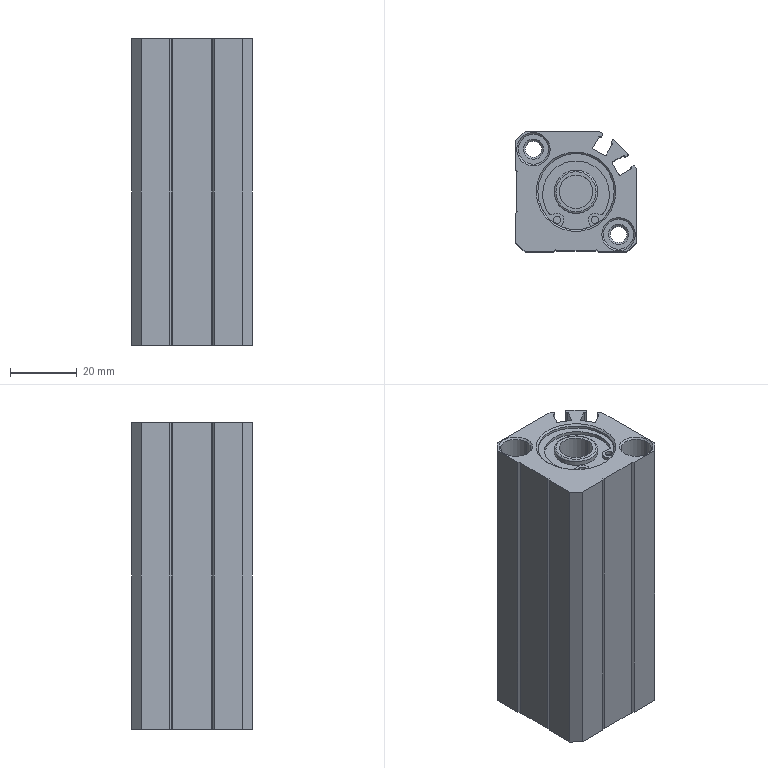Component | SolidWorks | ACQS_20x60_0-2_ACQS_20x6060_b-1 | 1 solid | 150 faces | volume 76906 mm3 | cylinder 68 | plane 52 | cone 28 | torus 2 | commonest cylinder face diameters 0.8 x14 9 x8 0.4 x6 20 x5 13 x4 1 x4 22.8 x4 4.134 x4